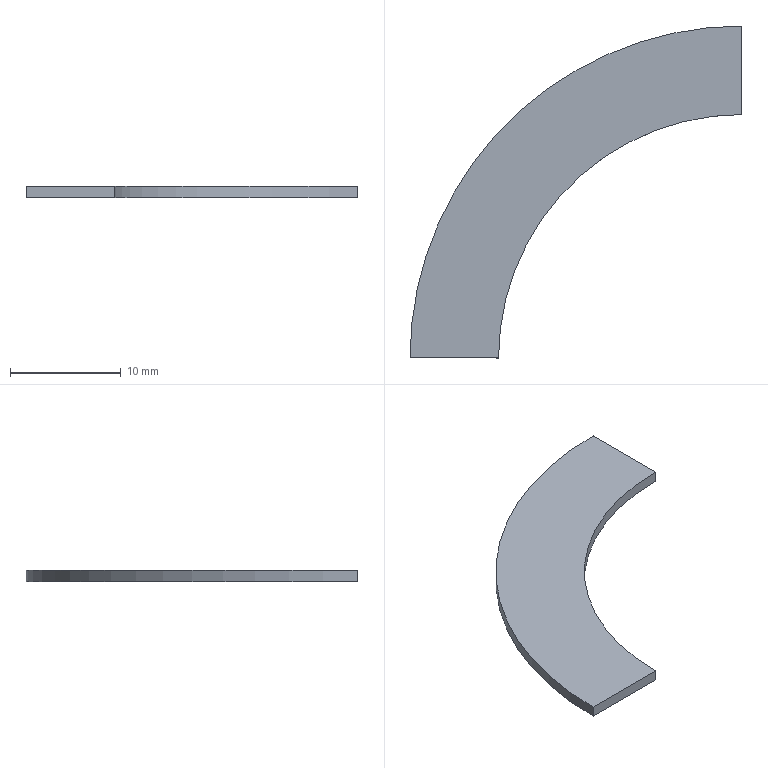Component | SolidWorks | Mirror_w5-2 | 1 solid | 6 faces | box 30 x 30 x 1 mm | volume 327 mm3 | plane 4 | cylinder 2 | commonest cylinder face diameters 44 x1 60 x1
STEP:
#1=CARTESIAN_POINT('',(-9.528,28.376,-1.378));
#2=VERTEX_POINT('',#1);
#3=CARTESIAN_POINT('',(-8.661,29.242,-1.378));
#4=VERTEX_POINT('',#3);
#5=CARTESIAN_POINT('',(-8.661,28.376,-1.378));
#6=DIRECTION('',(0.,0.,-1.));
#7=DIRECTION('',(1.,0.,0.));
#8=AXIS2_PLACEMENT_3D('',#5,#6,#7);
#9=CIRCLE('',#8,0.8661);
#10=EDGE_CURVE('',#2,#4,#9,.T.);
#11=ORIENTED_EDGE('',*,*,#10,.T.);
#12=CARTESIAN_POINT('',(-8.661,29.242,-1.339));
#13=VERTEX_POINT('',#12);
#14=CARTESIAN_POINT('',(-8.661,29.242,-1.339));
#15=DIRECTION('',(0.,0.,-1.));
#16=VECTOR('',#15,39.37);
#17=LINE('',#14,#16);
#18=EDGE_CURVE('',#13,#4,#17,.T.);
#19=ORIENTED_EDGE('',*,*,#18,.F.);
#20=CARTESIAN_POINT('',(-9.528,28.376,-1.339));
#21=VERTEX_POINT('',#20);
#22=CARTESIAN_POINT('',(-8.661,28.376,-1.339));
#23=DIRECTION('',(0.,0.,-1.));
#24=DIRECTION('',(1.,0.,0.));
#25=AXIS2_PLACEMENT_3D('',#22,#23,#24);
#26=CIRCLE('',#25,0.8661);
#27=EDGE_CURVE('',#21,#13,#26,.T.);
#28=ORIENTED_EDGE('',*,*,#27,.F.);
#29=CARTESIAN_POINT('',(-9.528,28.376,-1.339));
#30=DIRECTION('',(0.,0.,-1.));
#31=VECTOR('',#30,39.37);
#32=LINE('',#29,#31);
#33=EDGE_CURVE('',#21,#2,#32,.T.);
#34=ORIENTED_EDGE('',*,*,#33,.T.);
#35=EDGE_LOOP('',(#11,#19,#28,#34));
#36=FACE_OUTER_BOUND('',#35,.T.);
#37=CARTESIAN_POINT('',(-8.661,28.376,-1.339));
#38=DIRECTION('',(0.,0.,-1.));
#39=DIRECTION('',(1.,0.,0.));
#40=AXIS2_PLACEMENT_3D('',#37,#38,#39);
#41=CYLINDRICAL_SURFACE('',#40,0.8661);
#42=ADVANCED_FACE('',(#36),#41,.F.);
#43=CARTESIAN_POINT('',(-9.843,28.376,-1.378));
#44=VERTEX_POINT('',#43);
#45=CARTESIAN_POINT('',(-9.528,28.376,-1.378));
#46=DIRECTION('',(1.,-0.,0.));
#47=VECTOR('',#46,39.37);
#48=LINE('',#45,#47);
#49=EDGE_CURVE('',#44,#2,#48,.T.);
#50=ORIENTED_EDGE('',*,*,#49,.T.);
#51=ORIENTED_EDGE('',*,*,#33,.F.);
#52=CARTESIAN_POINT('',(-9.843,28.376,-1.339));
#53=VERTEX_POINT('',#52);
#54=CARTESIAN_POINT('',(-9.528,28.376,-1.339));
#55=DIRECTION('',(1.,-0.,0.));
#56=VECTOR('',#55,39.37);
#57=LINE('',#54,#56);
#58=EDGE_CURVE('',#53,#21,#57,.T.);
#59=ORIENTED_EDGE('',*,*,#58,.F.);
#60=CARTESIAN_POINT('',(-9.843,28.376,-1.339));
#61=DIRECTION('',(0.,0.,-1.));
#62=VECTOR('',#61,39.37);
#63=LINE('',#60,#62);
#64=EDGE_CURVE('',#53,#44,#63,.T.);
#65=ORIENTED_EDGE('',*,*,#64,.T.);
#66=EDGE_LOOP('',(#50,#51,#59,#65));
#67=FACE_OUTER_BOUND('',#66,.T.);
#68=CARTESIAN_POINT('',(-9.528,28.376,-1.339));
#69=DIRECTION('',(-0.,-1.,0.));
#70=DIRECTION('',(1.,-0.,0.));
#71=AXIS2_PLACEMENT_3D('',#68,#69,#70);
#72=PLANE('',#71);
#73=ADVANCED_FACE('',(#67),#72,.T.);
#74=CARTESIAN_POINT('',(-8.661,29.557,-1.378));
#75=VERTEX_POINT('',#74);
#76=CARTESIAN_POINT('',(-8.661,28.376,-1.378));
#77=DIRECTION('',(0.,0.,1.));
#78=DIRECTION('',(1.,0.,0.));
#79=AXIS2_PLACEMENT_3D('',#76,#77,#78);
#80=CIRCLE('',#79,1.181);
#81=EDGE_CURVE('',#75,#44,#80,.T.);
#82=ORIENTED_EDGE('',*,*,#81,.T.);
#83=ORIENTED_EDGE('',*,*,#64,.F.);
#84=CARTESIAN_POINT('',(-8.661,29.557,-1.339));
#85=VERTEX_POINT('',#84);
#86=CARTESIAN_POINT('',(-8.661,28.376,-1.339));
#87=DIRECTION('',(0.,0.,1.));
#88=DIRECTION('',(1.,0.,0.));
#89=AXIS2_PLACEMENT_3D('',#86,#87,#88);
#90=CIRCLE('',#89,1.181);
#91=EDGE_CURVE('',#85,#53,#90,.T.);
#92=ORIENTED_EDGE('',*,*,#91,.F.);
#93=CARTESIAN_POINT('',(-8.661,29.557,-1.339));
#94=DIRECTION('',(0.,0.,-1.));
#95=VECTOR('',#94,39.37);
#96=LINE('',#93,#95);
#97=EDGE_CURVE('',#85,#75,#96,.T.);
#98=ORIENTED_EDGE('',*,*,#97,.T.);
#99=EDGE_LOOP('',(#82,#83,#92,#98));
#100=FACE_OUTER_BOUND('',#99,.T.);
#101=CARTESIAN_POINT('',(-8.661,28.376,-1.339));
#102=DIRECTION('',(0.,0.,-1.));
#103=DIRECTION('',(1.,0.,0.));
#104=AXIS2_PLACEMENT_3D('',#101,#102,#103);
#105=CYLINDRICAL_SURFACE('',#104,1.181);
#106=ADVANCED_FACE('',(#100),#105,.T.);
#107=CARTESIAN_POINT('',(-8.661,29.242,-1.378));
#108=DIRECTION('',(0.,1.,0.));
#109=VECTOR('',#108,39.37);
#110=LINE('',#107,#109);
#111=EDGE_CURVE('',#4,#75,#110,.T.);
#112=ORIENTED_EDGE('',*,*,#111,.T.);
#113=ORIENTED_EDGE('',*,*,#97,.F.);
#114=CARTESIAN_POINT('',(-8.661,29.242,-1.339));
#115=DIRECTION('',(0.,1.,0.));
#116=VECTOR('',#115,39.37);
#117=LINE('',#114,#116);
#118=EDGE_CURVE('',#13,#85,#117,.T.);
#119=ORIENTED_EDGE('',*,*,#118,.F.);
#120=ORIENTED_EDGE('',*,*,#18,.T.);
#121=EDGE_LOOP('',(#112,#113,#119,#120));
#122=FACE_OUTER_BOUND('',#121,.T.);
#123=CARTESIAN_POINT('',(-8.661,29.242,-1.339));
#124=DIRECTION('',(1.,0.,0.));
#125=DIRECTION('',(0.,0.,1.));
#126=AXIS2_PLACEMENT_3D('',#123,#124,#125);
#127=PLANE('',#126);
#128=ADVANCED_FACE('',(#122),#127,.T.);
#129=ORIENTED_EDGE('',*,*,#27,.T.);
#130=ORIENTED_EDGE('',*,*,#118,.T.);
#131=ORIENTED_EDGE('',*,*,#91,.T.);
#132=ORIENTED_EDGE('',*,*,#58,.T.);
#133=EDGE_LOOP('',(#129,#130,#131,#132));
#134=FACE_OUTER_BOUND('',#133,.T.);
#135=CARTESIAN_POINT('',(-8.661,28.376,-1.339));
#136=DIRECTION('',(0.,0.,-1.));
#137=DIRECTION('',(1.,0.,0.));
#138=AXIS2_PLACEMENT_3D('',#135,#136,#137);
#139=PLANE('',#138);
#140=ADVANCED_FACE('',(#134),#139,.F.);
#141=ORIENTED_EDGE('',*,*,#10,.F.);
#142=ORIENTED_EDGE('',*,*,#49,.F.);
#143=ORIENTED_EDGE('',*,*,#81,.F.);
#144=ORIENTED_EDGE('',*,*,#111,.F.);
#145=EDGE_LOOP('',(#141,#142,#143,#144));
#146=FACE_OUTER_BOUND('',#145,.T.);
#147=CARTESIAN_POINT('',(-8.661,28.376,-1.378));
#148=DIRECTION('',(0.,0.,-1.));
#149=DIRECTION('',(1.,0.,0.));
#150=AXIS2_PLACEMENT_3D('',#147,#148,#149);
#151=PLANE('',#150);
#152=ADVANCED_FACE('',(#146),#151,.T.);
#153=CLOSED_SHELL('',(#42,#73,#106,#128,#140,#152));
#154=MANIFOLD_SOLID_BREP('',#153);
#155=CARTESIAN_POINT('',(0.,0.,0.));
#156=DIRECTION('',(0.,0.,1.));
#157=DIRECTION('',(1.,0.,0.));
#158=AXIS2_PLACEMENT_3D('',#155,#156,#157);
#159=(LENGTH_UNIT()NAMED_UNIT(*)SI_UNIT($,.METRE.));
#160=LENGTH_MEASURE_WITH_UNIT(LENGTH_MEASURE(0.0254),#159);
#161=DIMENSIONAL_EXPONENTS(1.,0.,0.,0.,0.,0.,0.);
#162=(CONVERSION_BASED_UNIT('',#160)LENGTH_UNIT()NAMED_UNIT(#161));
#163=UNCERTAINTY_MEASURE_WITH_UNIT(LENGTH_MEASURE(0.00001),#162,'','');
#164=(NAMED_UNIT(*)PLANE_ANGLE_UNIT()SI_UNIT($,.RADIAN.));
#165=(NAMED_UNIT(*)SI_UNIT($,.STERADIAN.)SOLID_ANGLE_UNIT());
#166=(GEOMETRIC_REPRESENTATION_CONTEXT(3)GLOBAL_UNCERTAINTY_ASSIGNED_CONTEXT((#163))GLOBAL_UNIT_ASSIGNED_CONTEXT((#162,#164,#165))REPRESENTATION_CONTEXT('',''));
#167=ADVANCED_BREP_SHAPE_REPRESENTATION('',(#154,#158),#166);
#168=COLOUR_RGB('',0.7922,0.8196,0.9333);
#169=FILL_AREA_STYLE_COLOUR('',#168);
#170=FILL_AREA_STYLE('',(#169));
#171=SURFACE_STYLE_FILL_AREA(#170);
#172=SURFACE_SIDE_STYLE('',(#171));
#173=SURFACE_STYLE_USAGE(.BOTH.,#172);
#174=PRESENTATION_STYLE_ASSIGNMENT((#173));
#175=STYLED_ITEM('',(#174),#154);
#176=PRESENTATION_LAYER_ASSIGNMENT('','',(#175));
#177=(LENGTH_UNIT()NAMED_UNIT(*)SI_UNIT($,.METRE.));
#178=LENGTH_MEASURE_WITH_UNIT(LENGTH_MEASURE(0.0254),#177);
#179=DIMENSIONAL_EXPONENTS(1.,0.,0.,0.,0.,0.,0.);
#180=(CONVERSION_BASED_UNIT('',#178)LENGTH_UNIT()NAMED_UNIT(#179));
#181=UNCERTAINTY_MEASURE_WITH_UNIT(LENGTH_MEASURE(0.00001),#180,'','');
#182=(NAMED_UNIT(*)PLANE_ANGLE_UNIT()SI_UNIT($,.RADIAN.));
#183=(NAMED_UNIT(*)SI_UNIT($,.STERADIAN.)SOLID_ANGLE_UNIT());
#184=(GEOMETRIC_REPRESENTATION_CONTEXT(3)GLOBAL_UNCERTAINTY_ASSIGNED_CONTEXT((#181))GLOBAL_UNIT_ASSIGNED_CONTEXT((#180,#182,#183))REPRESENTATION_CONTEXT('',''));
#185=MECHANICAL_DESIGN_GEOMETRIC_PRESENTATION_REPRESENTATION('',(#175),#184);